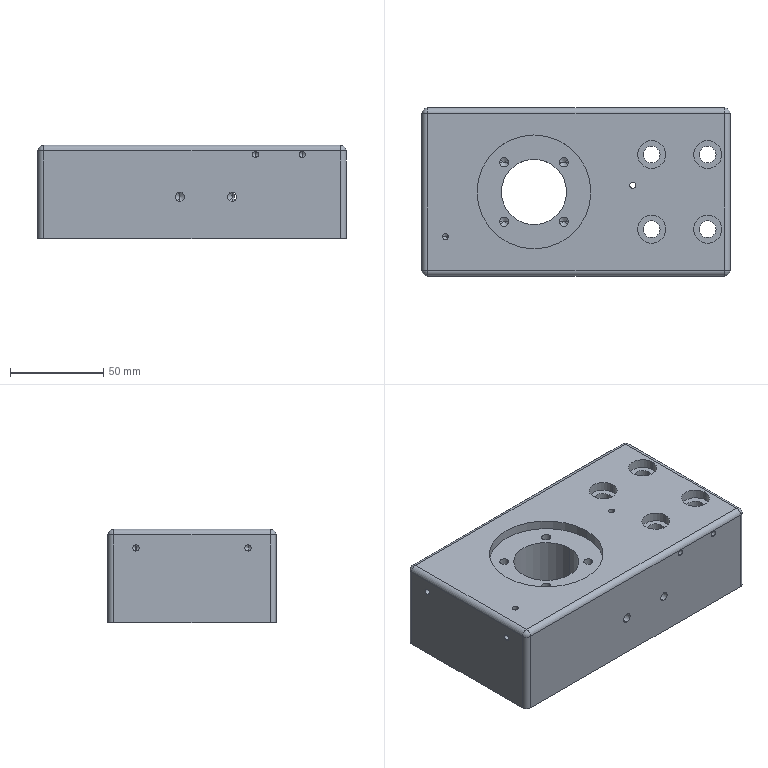Component | SolidWorks | ZDG0406-A03-P12-X1-1 | 1 solid | 130 faces | volume 471977 mm3 | cylinder 72 | cone 38 | plane 16 | sphere 4 | commonest cylinder face diameters 5 x24 3.3 x16 6 x10 15 x8 9 x8 61 x4 35 x2 | material 45#